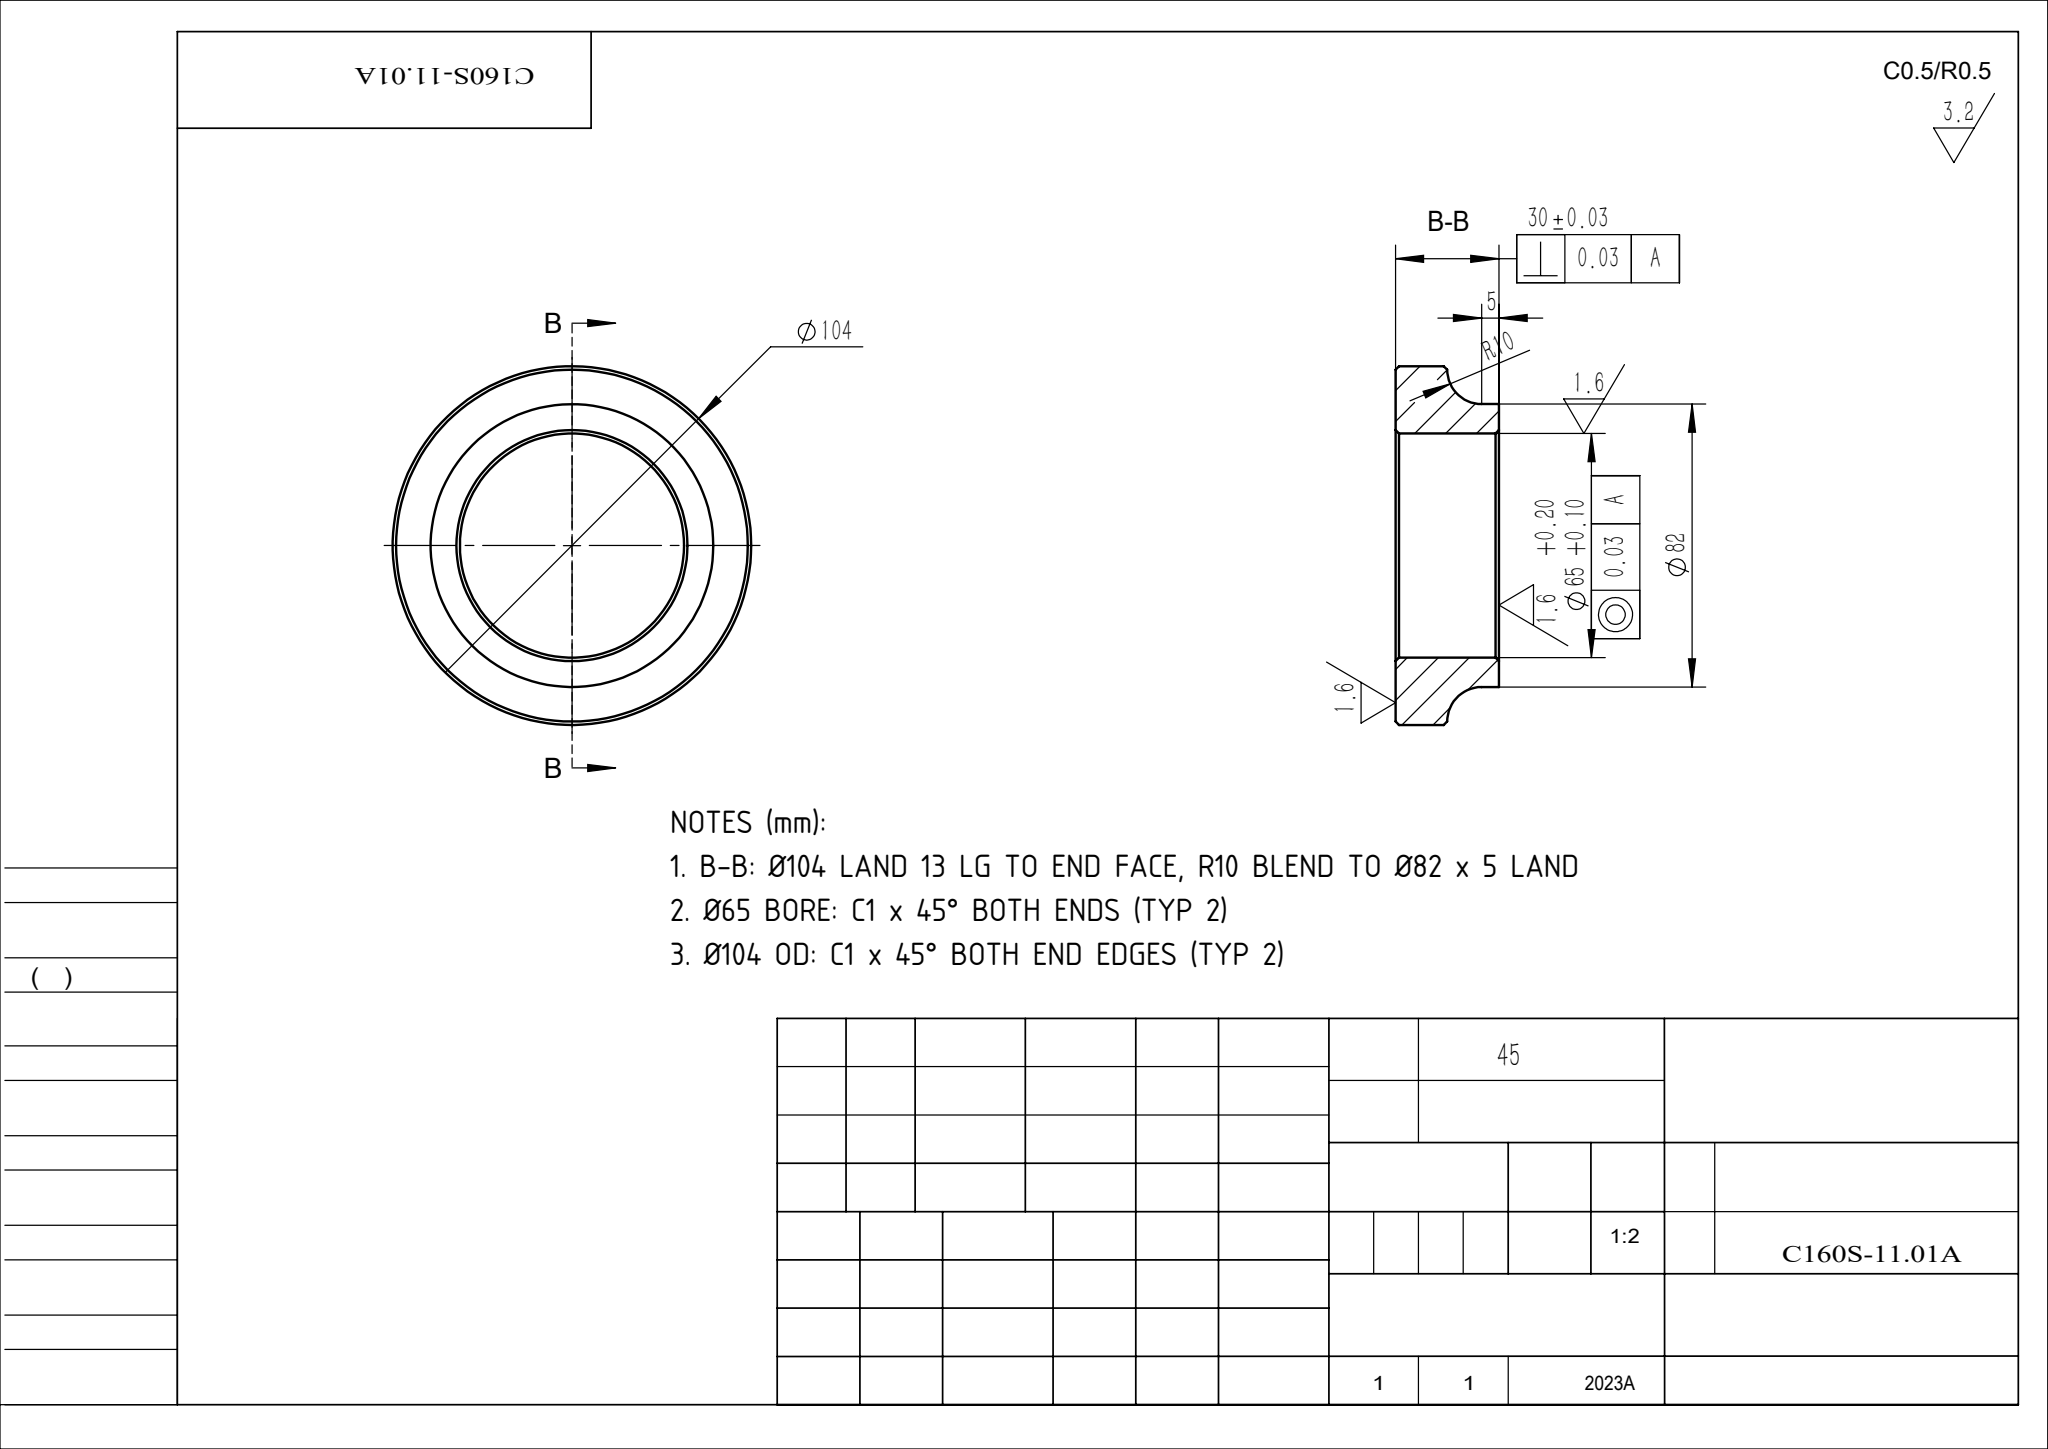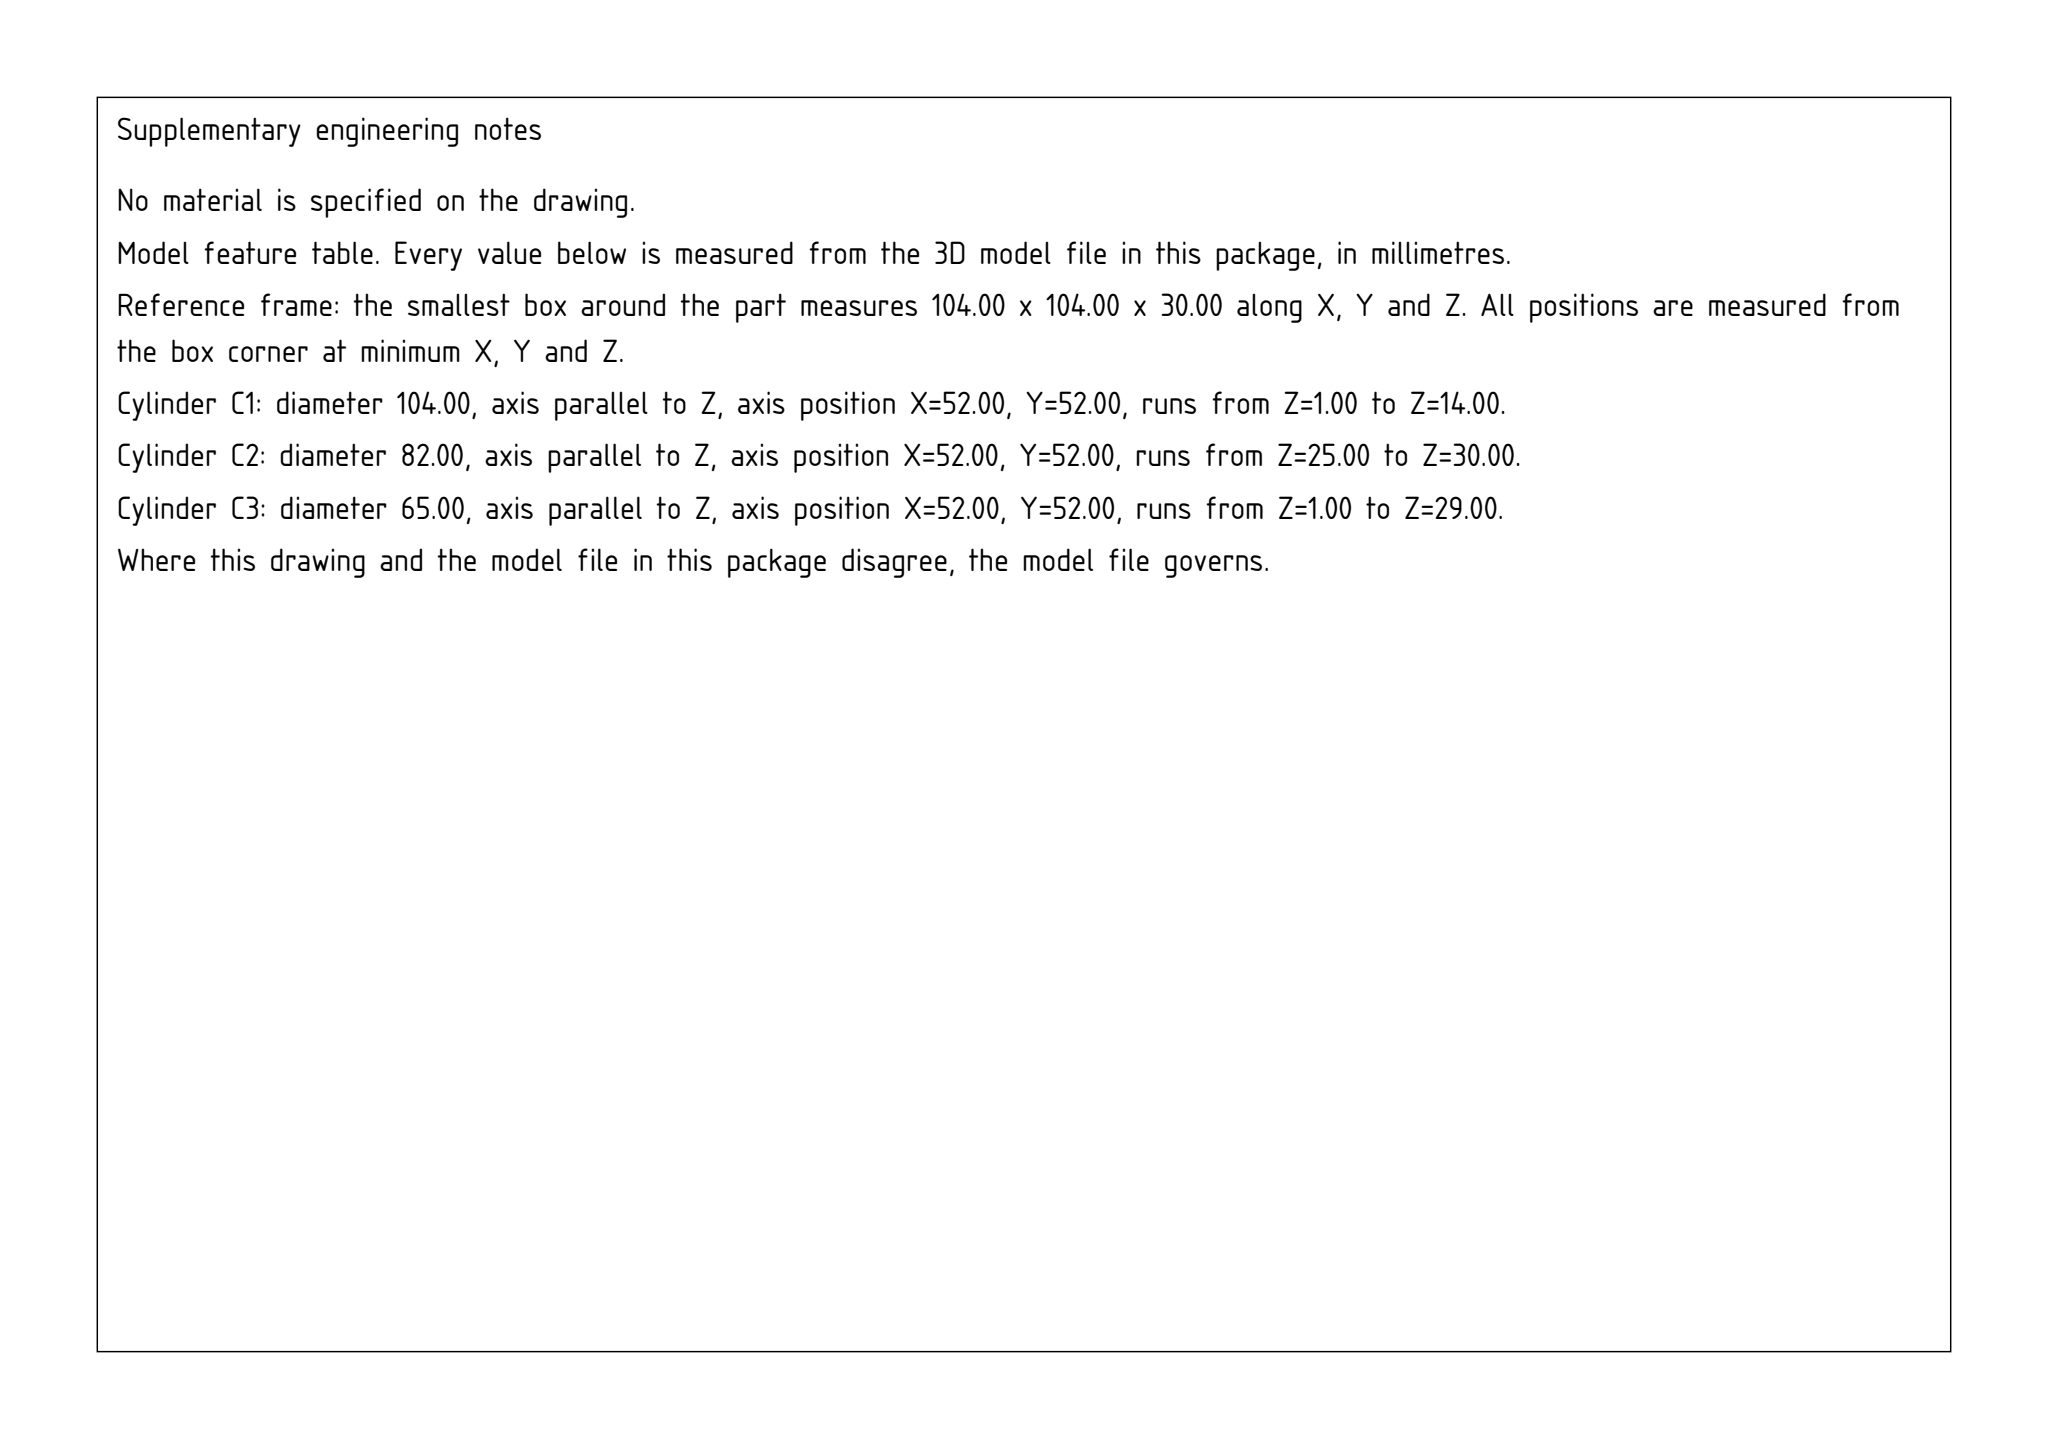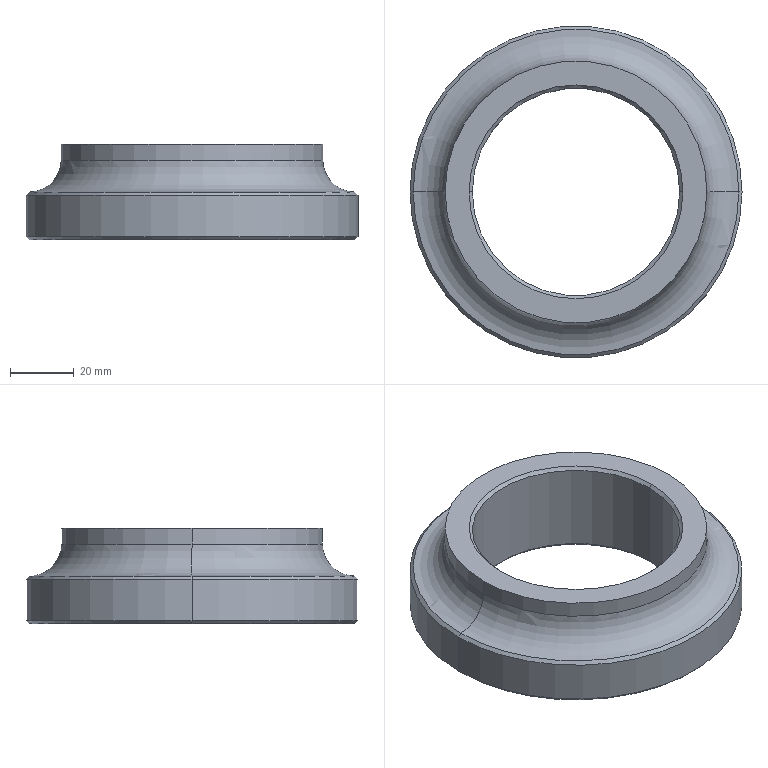Part | SolidWorks | mm | 1 solid | 18 faces | box 104 x 104 x 30 mm | volume 112388 mm3 | cone 8 | cylinder 6 | torus 2 | plane 2 | commonest cylinder face diameters 82 x2 65 x2 104 x2
Drawing notes:
B-B: Ø104 LAND 13 LG TO END FACE, R10 BLEND TO Ø82 x 5 LAND | from the solid: cyl Ø104 z-len 13; cyl Ø82 z-len 5; fillet R10; overall 30 (z-planes 0 & 30)
Ø65 BORE: C1 x 45° BOTH ENDS (TYP 2) | from the solid: cones 90° incl, ref dia 65 & 67 -> 1 mm x 45° chamfer, qty 2
Ø104 OD: C1 x 45° BOTH END EDGES (TYP 2) | from the solid: cones 90° incl, ref dia 102 & 104 -> 1 mm x 45° chamfer, qty 2
STEP:
#1=CARTESIAN_POINT('',(-41.,0.,25.));
#2=VERTEX_POINT('',#1);
#3=CARTESIAN_POINT('',(41.,0.,25.));
#4=VERTEX_POINT('',#3);
#5=CARTESIAN_POINT('',(0.,0.,25.));
#6=DIRECTION('',(0.,0.,1.));
#7=DIRECTION('',(1.,0.,0.));
#8=AXIS2_PLACEMENT_3D('',#5,#6,#7);
#9=CIRCLE('',#8,41.);
#10=EDGE_CURVE('',#2,#4,#9,.T.);
#11=ORIENTED_EDGE('',*,*,#10,.F.);
#12=CARTESIAN_POINT('',(-51.,0.,15.));
#13=VERTEX_POINT('',#12);
#14=CARTESIAN_POINT('',(-51.,0.,25.));
#15=DIRECTION('',(0.,1.,0.));
#16=DIRECTION('',(-1.,0.,0.));
#17=AXIS2_PLACEMENT_3D('',#14,#15,#16);
#18=CIRCLE('',#17,10.);
#19=EDGE_CURVE('',#2,#13,#18,.T.);
#20=ORIENTED_EDGE('',*,*,#19,.T.);
#21=CARTESIAN_POINT('',(51.,0.,15.));
#22=VERTEX_POINT('',#21);
#23=CARTESIAN_POINT('',(0.,0.,15.));
#24=DIRECTION('',(0.,0.,1.));
#25=DIRECTION('',(1.,0.,0.));
#26=AXIS2_PLACEMENT_3D('',#23,#24,#25);
#27=CIRCLE('',#26,51.);
#28=EDGE_CURVE('',#13,#22,#27,.T.);
#29=ORIENTED_EDGE('',*,*,#28,.T.);
#30=CARTESIAN_POINT('',(51.,0.,25.));
#31=DIRECTION('',(0.,-1.,0.));
#32=DIRECTION('',(0.,0.,-1.));
#33=AXIS2_PLACEMENT_3D('',#30,#31,#32);
#34=CIRCLE('',#33,10.);
#35=EDGE_CURVE('',#4,#22,#34,.T.);
#36=ORIENTED_EDGE('',*,*,#35,.F.);
#37=EDGE_LOOP('',(#11,#20,#29,#36));
#38=FACE_OUTER_BOUND('',#37,.T.);
#39=CARTESIAN_POINT('',(0.,0.,25.));
#40=DIRECTION('',(0.,0.,1.));
#41=DIRECTION('',(1.,0.,0.));
#42=AXIS2_PLACEMENT_3D('',#39,#40,#41);
#43=TOROIDAL_SURFACE('',#42,51.,10.);
#44=ADVANCED_FACE('',(#38),#43,.F.);
#45=CARTESIAN_POINT('',(0.,0.,15.));
#46=DIRECTION('',(0.,0.,1.));
#47=DIRECTION('',(1.,0.,0.));
#48=AXIS2_PLACEMENT_3D('',#45,#46,#47);
#49=CIRCLE('',#48,51.);
#50=EDGE_CURVE('',#22,#13,#49,.T.);
#51=ORIENTED_EDGE('',*,*,#50,.F.);
#52=CARTESIAN_POINT('',(52.,0.,14.));
#53=VERTEX_POINT('',#52);
#54=CARTESIAN_POINT('',(51.,0.,15.));
#55=DIRECTION('',(0.7071,0.,-0.7071));
#56=VECTOR('',#55,1000.);
#57=LINE('',#54,#56);
#58=EDGE_CURVE('',#22,#53,#57,.T.);
#59=ORIENTED_EDGE('',*,*,#58,.T.);
#60=CARTESIAN_POINT('',(-52.,0.,14.));
#61=VERTEX_POINT('',#60);
#62=CARTESIAN_POINT('',(0.,0.,14.));
#63=DIRECTION('',(0.,0.,-1.));
#64=DIRECTION('',(1.,0.,0.));
#65=AXIS2_PLACEMENT_3D('',#62,#63,#64);
#66=CIRCLE('',#65,52.);
#67=EDGE_CURVE('',#61,#53,#66,.T.);
#68=ORIENTED_EDGE('',*,*,#67,.F.);
#69=CARTESIAN_POINT('',(-51.,0.,15.));
#70=DIRECTION('',(-0.7071,0.,-0.7071));
#71=VECTOR('',#70,1000.);
#72=LINE('',#69,#71);
#73=EDGE_CURVE('',#13,#61,#72,.T.);
#74=ORIENTED_EDGE('',*,*,#73,.F.);
#75=EDGE_LOOP('',(#51,#59,#68,#74));
#76=FACE_OUTER_BOUND('',#75,.T.);
#77=CARTESIAN_POINT('',(0.,0.,15.));
#78=DIRECTION('',(0.,0.,-1.));
#79=DIRECTION('',(-1.,0.,0.));
#80=AXIS2_PLACEMENT_3D('',#77,#78,#79);
#81=CONICAL_SURFACE('',#80,51.,0.7854);
#82=ADVANCED_FACE('',(#76),#81,.T.);
#83=CARTESIAN_POINT('',(-51.,0.,0.));
#84=VERTEX_POINT('',#83);
#85=CARTESIAN_POINT('',(51.,0.,0.));
#86=VERTEX_POINT('',#85);
#87=CARTESIAN_POINT('',(0.,0.,0.));
#88=DIRECTION('',(0.,0.,-1.));
#89=DIRECTION('',(1.,0.,0.));
#90=AXIS2_PLACEMENT_3D('',#87,#88,#89);
#91=CIRCLE('',#90,51.);
#92=EDGE_CURVE('',#84,#86,#91,.T.);
#93=ORIENTED_EDGE('',*,*,#92,.F.);
#94=CARTESIAN_POINT('',(-52.,0.,1.));
#95=VERTEX_POINT('',#94);
#96=CARTESIAN_POINT('',(-52.,0.,1.));
#97=DIRECTION('',(-0.7071,0.,0.7071));
#98=VECTOR('',#97,1000.);
#99=LINE('',#96,#98);
#100=EDGE_CURVE('',#84,#95,#99,.T.);
#101=ORIENTED_EDGE('',*,*,#100,.T.);
#102=CARTESIAN_POINT('',(52.,0.,1.));
#103=VERTEX_POINT('',#102);
#104=CARTESIAN_POINT('',(0.,0.,1.));
#105=DIRECTION('',(0.,0.,1.));
#106=DIRECTION('',(1.,0.,0.));
#107=AXIS2_PLACEMENT_3D('',#104,#105,#106);
#108=CIRCLE('',#107,52.);
#109=EDGE_CURVE('',#103,#95,#108,.T.);
#110=ORIENTED_EDGE('',*,*,#109,.F.);
#111=CARTESIAN_POINT('',(52.,0.,1.));
#112=DIRECTION('',(0.7071,0.,0.7071));
#113=VECTOR('',#112,1000.);
#114=LINE('',#111,#113);
#115=EDGE_CURVE('',#86,#103,#114,.T.);
#116=ORIENTED_EDGE('',*,*,#115,.F.);
#117=EDGE_LOOP('',(#93,#101,#110,#116));
#118=FACE_OUTER_BOUND('',#117,.T.);
#119=CARTESIAN_POINT('',(0.,0.,1.));
#120=DIRECTION('',(0.,0.,1.));
#121=DIRECTION('',(1.,0.,0.));
#122=AXIS2_PLACEMENT_3D('',#119,#120,#121);
#123=CONICAL_SURFACE('',#122,52.,0.7854);
#124=ADVANCED_FACE('',(#118),#123,.T.);
#125=CARTESIAN_POINT('',(32.5,0.,1.));
#126=VERTEX_POINT('',#125);
#127=CARTESIAN_POINT('',(-32.5,0.,1.));
#128=VERTEX_POINT('',#127);
#129=CARTESIAN_POINT('',(0.,0.,1.));
#130=DIRECTION('',(0.,0.,-1.));
#131=DIRECTION('',(1.,0.,0.));
#132=AXIS2_PLACEMENT_3D('',#129,#130,#131);
#133=CIRCLE('',#132,32.5);
#134=EDGE_CURVE('',#126,#128,#133,.T.);
#135=ORIENTED_EDGE('',*,*,#134,.F.);
#136=CARTESIAN_POINT('',(33.5,0.,0.));
#137=VERTEX_POINT('',#136);
#138=CARTESIAN_POINT('',(33.5,0.,0.));
#139=DIRECTION('',(0.7071,0.,-0.7071));
#140=VECTOR('',#139,1000.);
#141=LINE('',#138,#140);
#142=EDGE_CURVE('',#126,#137,#141,.T.);
#143=ORIENTED_EDGE('',*,*,#142,.T.);
#144=CARTESIAN_POINT('',(-33.5,0.,0.));
#145=VERTEX_POINT('',#144);
#146=CARTESIAN_POINT('',(0.,0.,0.));
#147=DIRECTION('',(0.,0.,1.));
#148=DIRECTION('',(1.,0.,0.));
#149=AXIS2_PLACEMENT_3D('',#146,#147,#148);
#150=CIRCLE('',#149,33.5);
#151=EDGE_CURVE('',#145,#137,#150,.T.);
#152=ORIENTED_EDGE('',*,*,#151,.F.);
#153=CARTESIAN_POINT('',(-33.5,0.,0.));
#154=DIRECTION('',(-0.7071,0.,-0.7071));
#155=VECTOR('',#154,1000.);
#156=LINE('',#153,#155);
#157=EDGE_CURVE('',#128,#145,#156,.T.);
#158=ORIENTED_EDGE('',*,*,#157,.F.);
#159=EDGE_LOOP('',(#135,#143,#152,#158));
#160=FACE_OUTER_BOUND('',#159,.T.);
#161=CARTESIAN_POINT('',(0.,0.,0.));
#162=DIRECTION('',(0.,0.,-1.));
#163=DIRECTION('',(-1.,0.,0.));
#164=AXIS2_PLACEMENT_3D('',#161,#162,#163);
#165=CONICAL_SURFACE('',#164,33.5,0.7854);
#166=ADVANCED_FACE('',(#160),#165,.F.);
#167=CARTESIAN_POINT('',(-32.5,0.,29.));
#168=VERTEX_POINT('',#167);
#169=CARTESIAN_POINT('',(32.5,0.,29.));
#170=VERTEX_POINT('',#169);
#171=CARTESIAN_POINT('',(0.,0.,29.));
#172=DIRECTION('',(0.,0.,1.));
#173=DIRECTION('',(1.,0.,0.));
#174=AXIS2_PLACEMENT_3D('',#171,#172,#173);
#175=CIRCLE('',#174,32.5);
#176=EDGE_CURVE('',#168,#170,#175,.T.);
#177=ORIENTED_EDGE('',*,*,#176,.F.);
#178=CARTESIAN_POINT('',(-33.5,0.,30.));
#179=VERTEX_POINT('',#178);
#180=CARTESIAN_POINT('',(-32.5,0.,29.));
#181=DIRECTION('',(-0.7071,0.,0.7071));
#182=VECTOR('',#181,1000.);
#183=LINE('',#180,#182);
#184=EDGE_CURVE('',#168,#179,#183,.T.);
#185=ORIENTED_EDGE('',*,*,#184,.T.);
#186=CARTESIAN_POINT('',(33.5,0.,30.));
#187=VERTEX_POINT('',#186);
#188=CARTESIAN_POINT('',(0.,0.,30.));
#189=DIRECTION('',(0.,0.,-1.));
#190=DIRECTION('',(1.,0.,0.));
#191=AXIS2_PLACEMENT_3D('',#188,#189,#190);
#192=CIRCLE('',#191,33.5);
#193=EDGE_CURVE('',#187,#179,#192,.T.);
#194=ORIENTED_EDGE('',*,*,#193,.F.);
#195=CARTESIAN_POINT('',(32.5,0.,29.));
#196=DIRECTION('',(0.7071,0.,0.7071));
#197=VECTOR('',#196,1000.);
#198=LINE('',#195,#197);
#199=EDGE_CURVE('',#170,#187,#198,.T.);
#200=ORIENTED_EDGE('',*,*,#199,.F.);
#201=EDGE_LOOP('',(#177,#185,#194,#200));
#202=FACE_OUTER_BOUND('',#201,.T.);
#203=CARTESIAN_POINT('',(0.,0.,29.));
#204=DIRECTION('',(0.,0.,1.));
#205=DIRECTION('',(1.,0.,0.));
#206=AXIS2_PLACEMENT_3D('',#203,#204,#205);
#207=CONICAL_SURFACE('',#206,32.5,0.7854);
#208=ADVANCED_FACE('',(#202),#207,.F.);
#209=CARTESIAN_POINT('',(41.,0.,30.));
#210=VERTEX_POINT('',#209);
#211=CARTESIAN_POINT('',(-41.,0.,30.));
#212=VERTEX_POINT('',#211);
#213=CARTESIAN_POINT('',(0.,0.,30.));
#214=DIRECTION('',(0.,0.,1.));
#215=DIRECTION('',(1.,0.,0.));
#216=AXIS2_PLACEMENT_3D('',#213,#214,#215);
#217=CIRCLE('',#216,41.);
#218=EDGE_CURVE('',#210,#212,#217,.T.);
#219=ORIENTED_EDGE('',*,*,#218,.F.);
#220=CARTESIAN_POINT('',(41.,0.,30.));
#221=DIRECTION('',(0.,0.,-1.));
#222=VECTOR('',#221,1000.);
#223=LINE('',#220,#222);
#224=EDGE_CURVE('',#210,#4,#223,.T.);
#225=ORIENTED_EDGE('',*,*,#224,.T.);
#226=CARTESIAN_POINT('',(0.,0.,25.));
#227=DIRECTION('',(0.,0.,1.));
#228=DIRECTION('',(1.,0.,0.));
#229=AXIS2_PLACEMENT_3D('',#226,#227,#228);
#230=CIRCLE('',#229,41.);
#231=EDGE_CURVE('',#4,#2,#230,.T.);
#232=ORIENTED_EDGE('',*,*,#231,.T.);
#233=CARTESIAN_POINT('',(-41.,0.,30.));
#234=DIRECTION('',(0.,0.,-1.));
#235=VECTOR('',#234,1000.);
#236=LINE('',#233,#235);
#237=EDGE_CURVE('',#212,#2,#236,.T.);
#238=ORIENTED_EDGE('',*,*,#237,.F.);
#239=EDGE_LOOP('',(#219,#225,#232,#238));
#240=FACE_OUTER_BOUND('',#239,.T.);
#241=CARTESIAN_POINT('',(0.,0.,30.));
#242=DIRECTION('',(0.,0.,-1.));
#243=DIRECTION('',(-1.,0.,0.));
#244=AXIS2_PLACEMENT_3D('',#241,#242,#243);
#245=CYLINDRICAL_SURFACE('',#244,41.);
#246=ADVANCED_FACE('',(#240),#245,.T.);
#247=ORIENTED_EDGE('',*,*,#176,.T.);
#248=CARTESIAN_POINT('',(32.5,0.,15.));
#249=DIRECTION('',(0.,0.,-1.));
#250=VECTOR('',#249,1000.);
#251=LINE('',#248,#250);
#252=EDGE_CURVE('',#170,#126,#251,.T.);
#253=ORIENTED_EDGE('',*,*,#252,.T.);
#254=ORIENTED_EDGE('',*,*,#134,.T.);
#255=CARTESIAN_POINT('',(-32.5,0.,15.));
#256=DIRECTION('',(0.,0.,-1.));
#257=VECTOR('',#256,1000.);
#258=LINE('',#255,#257);
#259=EDGE_CURVE('',#168,#128,#258,.T.);
#260=ORIENTED_EDGE('',*,*,#259,.F.);
#261=EDGE_LOOP('',(#247,#253,#254,#260));
#262=FACE_OUTER_BOUND('',#261,.T.);
#263=CARTESIAN_POINT('',(0.,0.,15.));
#264=DIRECTION('',(0.,0.,-1.));
#265=DIRECTION('',(-1.,0.,0.));
#266=AXIS2_PLACEMENT_3D('',#263,#264,#265);
#267=CYLINDRICAL_SURFACE('',#266,32.5);
#268=ADVANCED_FACE('',(#262),#267,.F.);
#269=ORIENTED_EDGE('',*,*,#67,.T.);
#270=CARTESIAN_POINT('',(52.,0.,15.));
#271=DIRECTION('',(0.,0.,-1.));
#272=VECTOR('',#271,1000.);
#273=LINE('',#270,#272);
#274=EDGE_CURVE('',#53,#103,#273,.T.);
#275=ORIENTED_EDGE('',*,*,#274,.T.);
#276=ORIENTED_EDGE('',*,*,#109,.T.);
#277=CARTESIAN_POINT('',(-52.,0.,15.));
#278=DIRECTION('',(0.,0.,-1.));
#279=VECTOR('',#278,1000.);
#280=LINE('',#277,#279);
#281=EDGE_CURVE('',#61,#95,#280,.T.);
#282=ORIENTED_EDGE('',*,*,#281,.F.);
#283=EDGE_LOOP('',(#269,#275,#276,#282));
#284=FACE_OUTER_BOUND('',#283,.T.);
#285=CARTESIAN_POINT('',(0.,0.,15.));
#286=DIRECTION('',(0.,0.,-1.));
#287=DIRECTION('',(-1.,0.,0.));
#288=AXIS2_PLACEMENT_3D('',#285,#286,#287);
#289=CYLINDRICAL_SURFACE('',#288,52.);
#290=ADVANCED_FACE('',(#284),#289,.T.);
#291=ORIENTED_EDGE('',*,*,#151,.T.);
#292=CARTESIAN_POINT('',(0.,0.,0.));
#293=DIRECTION('',(0.,0.,1.));
#294=DIRECTION('',(1.,0.,0.));
#295=AXIS2_PLACEMENT_3D('',#292,#293,#294);
#296=CIRCLE('',#295,33.5);
#297=EDGE_CURVE('',#137,#145,#296,.T.);
#298=ORIENTED_EDGE('',*,*,#297,.T.);
#299=EDGE_LOOP('',(#291,#298));
#300=FACE_BOUND('',#299,.T.);
#301=CARTESIAN_POINT('',(0.,0.,0.));
#302=DIRECTION('',(0.,0.,-1.));
#303=DIRECTION('',(1.,0.,0.));
#304=AXIS2_PLACEMENT_3D('',#301,#302,#303);
#305=CIRCLE('',#304,51.);
#306=EDGE_CURVE('',#86,#84,#305,.T.);
#307=ORIENTED_EDGE('',*,*,#306,.T.);
#308=ORIENTED_EDGE('',*,*,#92,.T.);
#309=EDGE_LOOP('',(#307,#308));
#310=FACE_OUTER_BOUND('',#309,.T.);
#311=CARTESIAN_POINT('',(0.,0.,0.));
#312=DIRECTION('',(0.,0.,1.));
#313=DIRECTION('',(1.,0.,0.));
#314=AXIS2_PLACEMENT_3D('',#311,#312,#313);
#315=PLANE('',#314);
#316=ADVANCED_FACE('',(#300,#310),#315,.F.);
#317=ORIENTED_EDGE('',*,*,#274,.F.);
#318=CARTESIAN_POINT('',(0.,0.,14.));
#319=DIRECTION('',(0.,0.,-1.));
#320=DIRECTION('',(1.,0.,0.));
#321=AXIS2_PLACEMENT_3D('',#318,#319,#320);
#322=CIRCLE('',#321,52.);
#323=EDGE_CURVE('',#53,#61,#322,.T.);
#324=ORIENTED_EDGE('',*,*,#323,.T.);
#325=ORIENTED_EDGE('',*,*,#281,.T.);
#326=CARTESIAN_POINT('',(0.,0.,1.));
#327=DIRECTION('',(0.,0.,1.));
#328=DIRECTION('',(1.,0.,0.));
#329=AXIS2_PLACEMENT_3D('',#326,#327,#328);
#330=CIRCLE('',#329,52.);
#331=EDGE_CURVE('',#95,#103,#330,.T.);
#332=ORIENTED_EDGE('',*,*,#331,.T.);
#333=EDGE_LOOP('',(#317,#324,#325,#332));
#334=FACE_OUTER_BOUND('',#333,.T.);
#335=CARTESIAN_POINT('',(0.,0.,15.));
#336=DIRECTION('',(0.,0.,-1.));
#337=DIRECTION('',(-1.,0.,0.));
#338=AXIS2_PLACEMENT_3D('',#335,#336,#337);
#339=CYLINDRICAL_SURFACE('',#338,52.);
#340=ADVANCED_FACE('',(#334),#339,.T.);
#341=ORIENTED_EDGE('',*,*,#252,.F.);
#342=CARTESIAN_POINT('',(0.,0.,29.));
#343=DIRECTION('',(0.,0.,1.));
#344=DIRECTION('',(1.,0.,0.));
#345=AXIS2_PLACEMENT_3D('',#342,#343,#344);
#346=CIRCLE('',#345,32.5);
#347=EDGE_CURVE('',#170,#168,#346,.T.);
#348=ORIENTED_EDGE('',*,*,#347,.T.);
#349=ORIENTED_EDGE('',*,*,#259,.T.);
#350=CARTESIAN_POINT('',(0.,0.,1.));
#351=DIRECTION('',(0.,0.,-1.));
#352=DIRECTION('',(1.,0.,0.));
#353=AXIS2_PLACEMENT_3D('',#350,#351,#352);
#354=CIRCLE('',#353,32.5);
#355=EDGE_CURVE('',#128,#126,#354,.T.);
#356=ORIENTED_EDGE('',*,*,#355,.T.);
#357=EDGE_LOOP('',(#341,#348,#349,#356));
#358=FACE_OUTER_BOUND('',#357,.T.);
#359=CARTESIAN_POINT('',(0.,0.,15.));
#360=DIRECTION('',(0.,0.,-1.));
#361=DIRECTION('',(-1.,0.,0.));
#362=AXIS2_PLACEMENT_3D('',#359,#360,#361);
#363=CYLINDRICAL_SURFACE('',#362,32.5);
#364=ADVANCED_FACE('',(#358),#363,.F.);
#365=ORIENTED_EDGE('',*,*,#193,.T.);
#366=CARTESIAN_POINT('',(0.,0.,30.));
#367=DIRECTION('',(0.,0.,-1.));
#368=DIRECTION('',(1.,0.,0.));
#369=AXIS2_PLACEMENT_3D('',#366,#367,#368);
#370=CIRCLE('',#369,33.5);
#371=EDGE_CURVE('',#179,#187,#370,.T.);
#372=ORIENTED_EDGE('',*,*,#371,.T.);
#373=EDGE_LOOP('',(#365,#372));
#374=FACE_BOUND('',#373,.T.);
#375=CARTESIAN_POINT('',(0.,0.,30.));
#376=DIRECTION('',(0.,0.,1.));
#377=DIRECTION('',(1.,0.,0.));
#378=AXIS2_PLACEMENT_3D('',#375,#376,#377);
#379=CIRCLE('',#378,41.);
#380=EDGE_CURVE('',#212,#210,#379,.T.);
#381=ORIENTED_EDGE('',*,*,#380,.T.);
#382=ORIENTED_EDGE('',*,*,#218,.T.);
#383=EDGE_LOOP('',(#381,#382));
#384=FACE_OUTER_BOUND('',#383,.T.);
#385=CARTESIAN_POINT('',(0.,0.,30.));
#386=DIRECTION('',(0.,0.,1.));
#387=DIRECTION('',(1.,0.,0.));
#388=AXIS2_PLACEMENT_3D('',#385,#386,#387);
#389=PLANE('',#388);
#390=ADVANCED_FACE('',(#374,#384),#389,.T.);
#391=ORIENTED_EDGE('',*,*,#224,.F.);
#392=ORIENTED_EDGE('',*,*,#380,.F.);
#393=ORIENTED_EDGE('',*,*,#237,.T.);
#394=ORIENTED_EDGE('',*,*,#10,.T.);
#395=EDGE_LOOP('',(#391,#392,#393,#394));
#396=FACE_OUTER_BOUND('',#395,.T.);
#397=CARTESIAN_POINT('',(0.,0.,30.));
#398=DIRECTION('',(0.,0.,-1.));
#399=DIRECTION('',(-1.,0.,0.));
#400=AXIS2_PLACEMENT_3D('',#397,#398,#399);
#401=CYLINDRICAL_SURFACE('',#400,41.);
#402=ADVANCED_FACE('',(#396),#401,.T.);
#403=ORIENTED_EDGE('',*,*,#184,.F.);
#404=ORIENTED_EDGE('',*,*,#347,.F.);
#405=ORIENTED_EDGE('',*,*,#199,.T.);
#406=ORIENTED_EDGE('',*,*,#371,.F.);
#407=EDGE_LOOP('',(#403,#404,#405,#406));
#408=FACE_OUTER_BOUND('',#407,.T.);
#409=CARTESIAN_POINT('',(0.,0.,29.));
#410=DIRECTION('',(0.,0.,1.));
#411=DIRECTION('',(1.,0.,0.));
#412=AXIS2_PLACEMENT_3D('',#409,#410,#411);
#413=CONICAL_SURFACE('',#412,32.5,0.7854);
#414=ADVANCED_FACE('',(#408),#413,.F.);
#415=ORIENTED_EDGE('',*,*,#142,.F.);
#416=ORIENTED_EDGE('',*,*,#355,.F.);
#417=ORIENTED_EDGE('',*,*,#157,.T.);
#418=ORIENTED_EDGE('',*,*,#297,.F.);
#419=EDGE_LOOP('',(#415,#416,#417,#418));
#420=FACE_OUTER_BOUND('',#419,.T.);
#421=CARTESIAN_POINT('',(0.,0.,0.));
#422=DIRECTION('',(0.,0.,-1.));
#423=DIRECTION('',(-1.,0.,0.));
#424=AXIS2_PLACEMENT_3D('',#421,#422,#423);
#425=CONICAL_SURFACE('',#424,33.5,0.7854);
#426=ADVANCED_FACE('',(#420),#425,.F.);
#427=ORIENTED_EDGE('',*,*,#100,.F.);
#428=ORIENTED_EDGE('',*,*,#306,.F.);
#429=ORIENTED_EDGE('',*,*,#115,.T.);
#430=ORIENTED_EDGE('',*,*,#331,.F.);
#431=EDGE_LOOP('',(#427,#428,#429,#430));
#432=FACE_OUTER_BOUND('',#431,.T.);
#433=CARTESIAN_POINT('',(0.,0.,1.));
#434=DIRECTION('',(0.,0.,1.));
#435=DIRECTION('',(1.,0.,0.));
#436=AXIS2_PLACEMENT_3D('',#433,#434,#435);
#437=CONICAL_SURFACE('',#436,52.,0.7854);
#438=ADVANCED_FACE('',(#432),#437,.T.);
#439=ORIENTED_EDGE('',*,*,#58,.F.);
#440=ORIENTED_EDGE('',*,*,#28,.F.);
#441=ORIENTED_EDGE('',*,*,#73,.T.);
#442=ORIENTED_EDGE('',*,*,#323,.F.);
#443=EDGE_LOOP('',(#439,#440,#441,#442));
#444=FACE_OUTER_BOUND('',#443,.T.);
#445=CARTESIAN_POINT('',(0.,0.,15.));
#446=DIRECTION('',(0.,0.,-1.));
#447=DIRECTION('',(-1.,0.,0.));
#448=AXIS2_PLACEMENT_3D('',#445,#446,#447);
#449=CONICAL_SURFACE('',#448,51.,0.7854);
#450=ADVANCED_FACE('',(#444),#449,.T.);
#451=ORIENTED_EDGE('',*,*,#19,.F.);
#452=ORIENTED_EDGE('',*,*,#231,.F.);
#453=ORIENTED_EDGE('',*,*,#35,.T.);
#454=ORIENTED_EDGE('',*,*,#50,.T.);
#455=EDGE_LOOP('',(#451,#452,#453,#454));
#456=FACE_OUTER_BOUND('',#455,.T.);
#457=CARTESIAN_POINT('',(0.,0.,25.));
#458=DIRECTION('',(0.,0.,1.));
#459=DIRECTION('',(1.,0.,0.));
#460=AXIS2_PLACEMENT_3D('',#457,#458,#459);
#461=TOROIDAL_SURFACE('',#460,51.,10.);
#462=ADVANCED_FACE('',(#456),#461,.F.);
#463=CLOSED_SHELL('',(#44,#82,#124,#166,#208,#246,#268,#290,#316,#340,#364,#390,#402,#414,#426,#438,#450,#462));
#464=MANIFOLD_SOLID_BREP('',#463);
#465=CARTESIAN_POINT('',(0.,0.,0.));
#466=DIRECTION('',(0.,0.,1.));
#467=DIRECTION('',(1.,0.,0.));
#468=AXIS2_PLACEMENT_3D('',#465,#466,#467);
#469=(LENGTH_UNIT()NAMED_UNIT(*)SI_UNIT(.MILLI.,.METRE.));
#470=UNCERTAINTY_MEASURE_WITH_UNIT(LENGTH_MEASURE(0.00001),#469,'','');
#471=(NAMED_UNIT(*)PLANE_ANGLE_UNIT()SI_UNIT($,.RADIAN.));
#472=(NAMED_UNIT(*)SI_UNIT($,.STERADIAN.)SOLID_ANGLE_UNIT());
#473=(GEOMETRIC_REPRESENTATION_CONTEXT(3)GLOBAL_UNCERTAINTY_ASSIGNED_CONTEXT((#470))GLOBAL_UNIT_ASSIGNED_CONTEXT((#469,#471,#472))REPRESENTATION_CONTEXT('',''));
#474=ADVANCED_BREP_SHAPE_REPRESENTATION('',(#464,#468),#473);